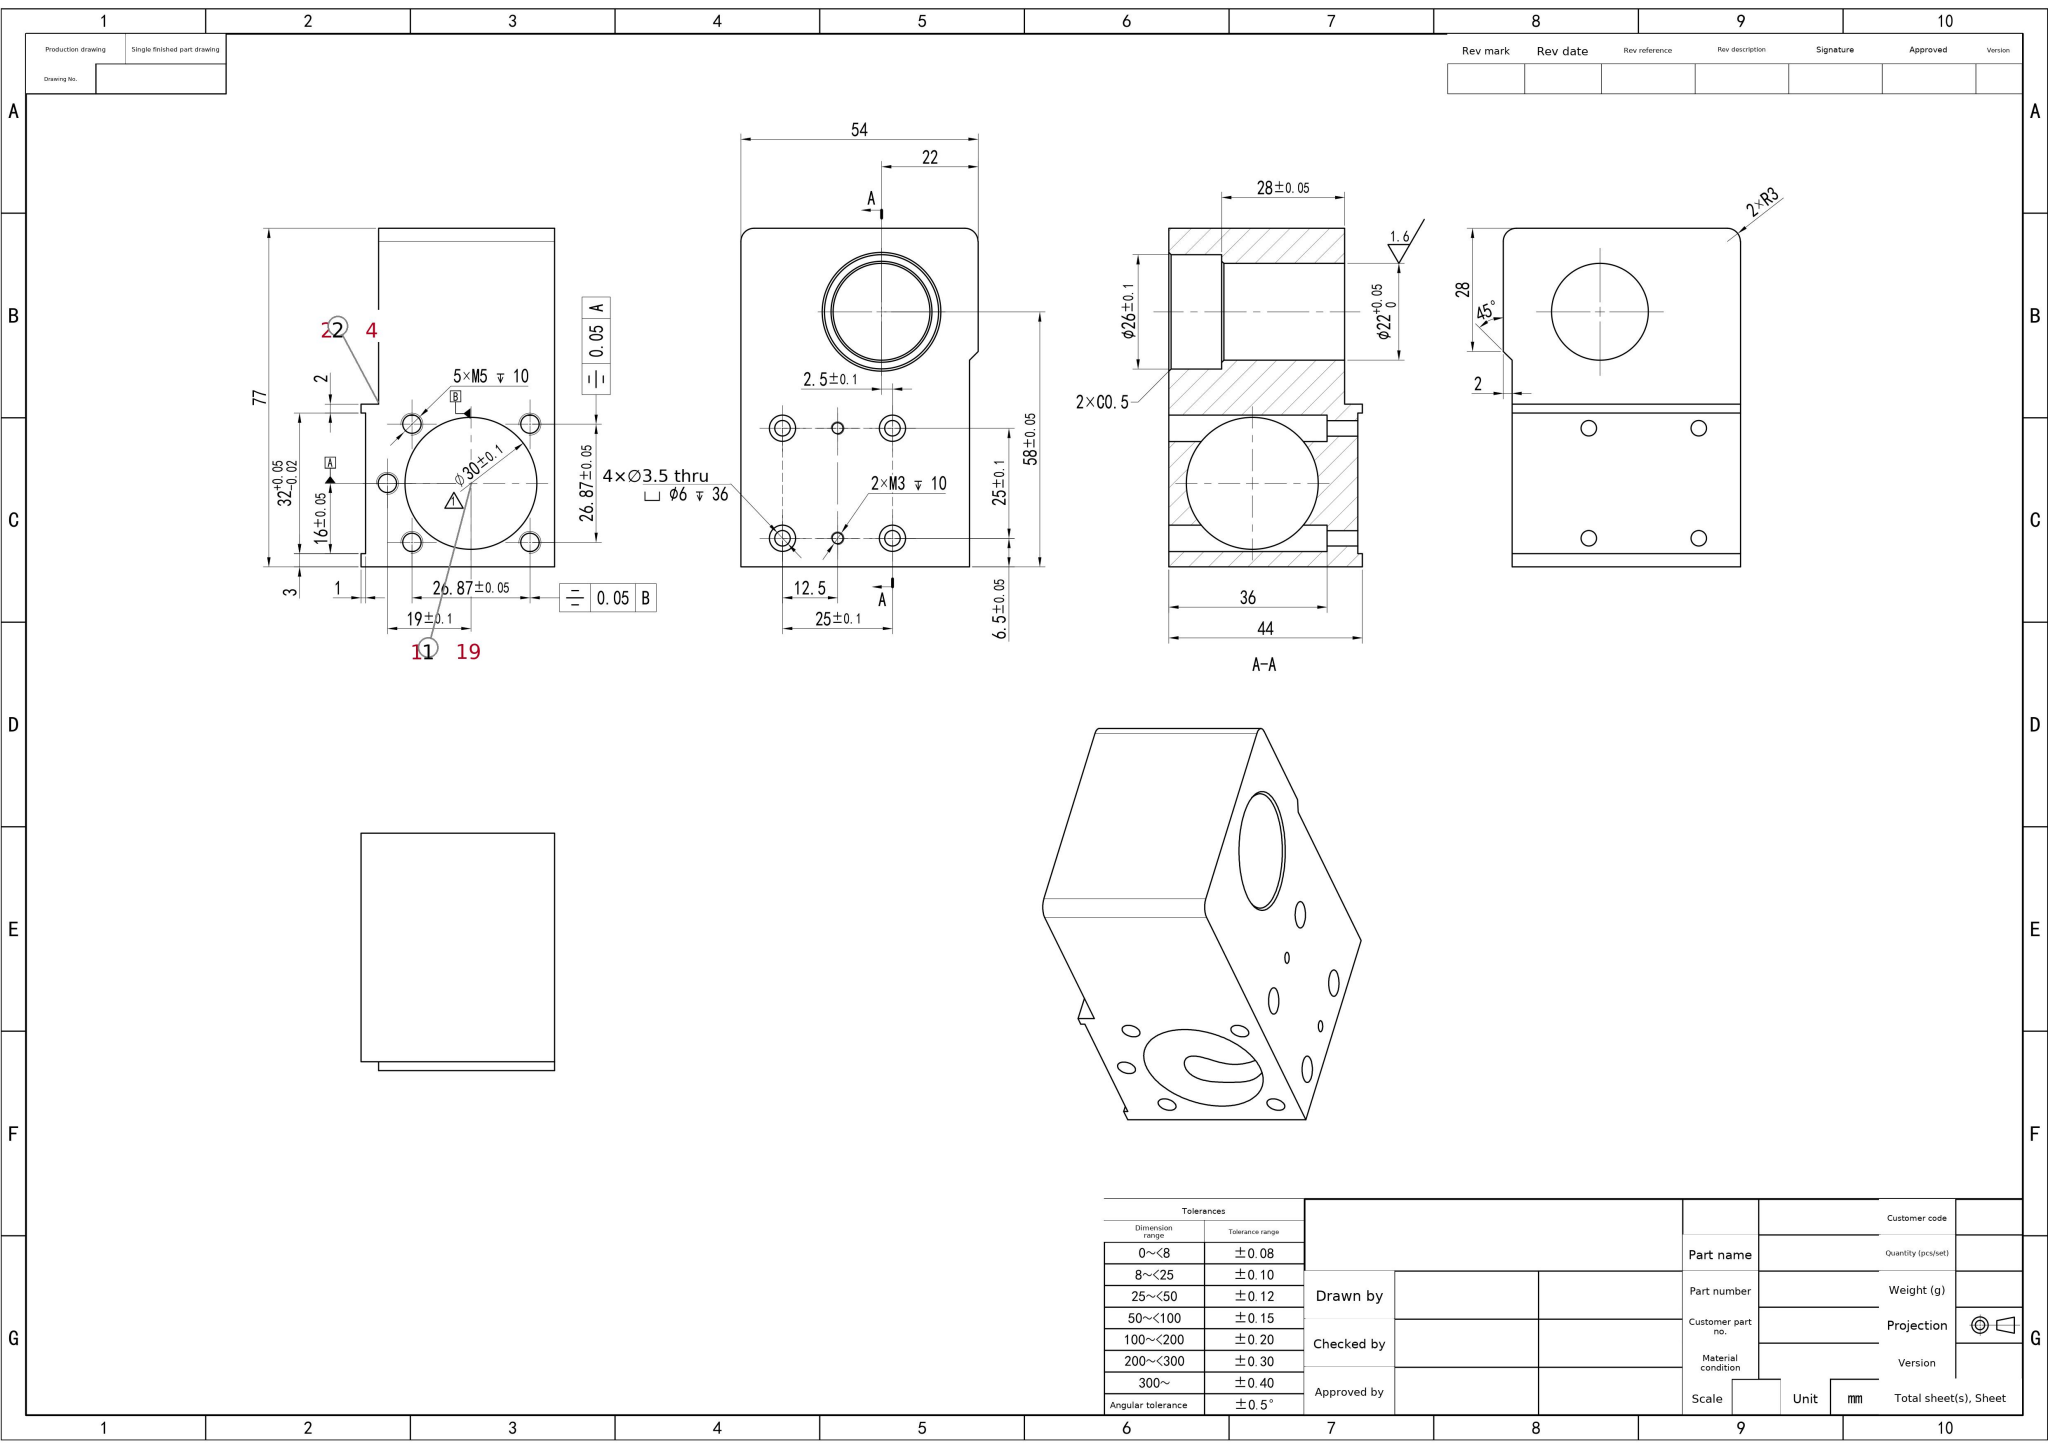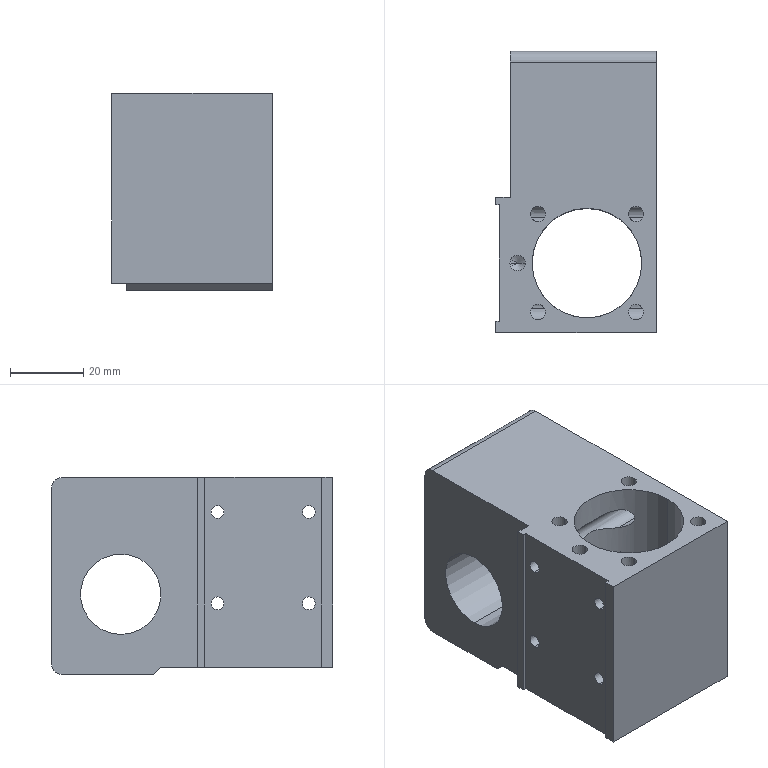Part | SolidWorks | mm | 1 solid | 77 faces | box 44 x 77 x 54 mm | volume 111332 mm3 | cylinder 42 | plane 19 | cone 16 | commonest cylinder face diameters 6 x14 4.2 x10 3.5 x8 2.5 x4 30 x2 22 x2 26 x2